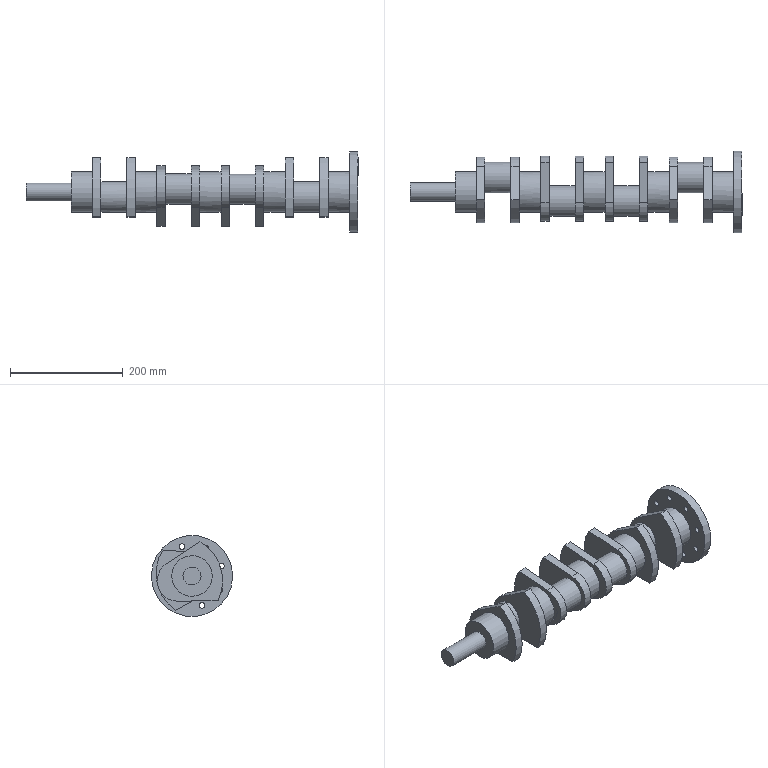Component | NX | 7_CRANKSHAFT | 5 solids | 90 faces | volume 2580901 mm3 | plane 48 | cylinder 42 | commonest cylinder face diameters 72 x13 54 x8 160 x8 10 x8 53.987 x3 32 x1 144 x1